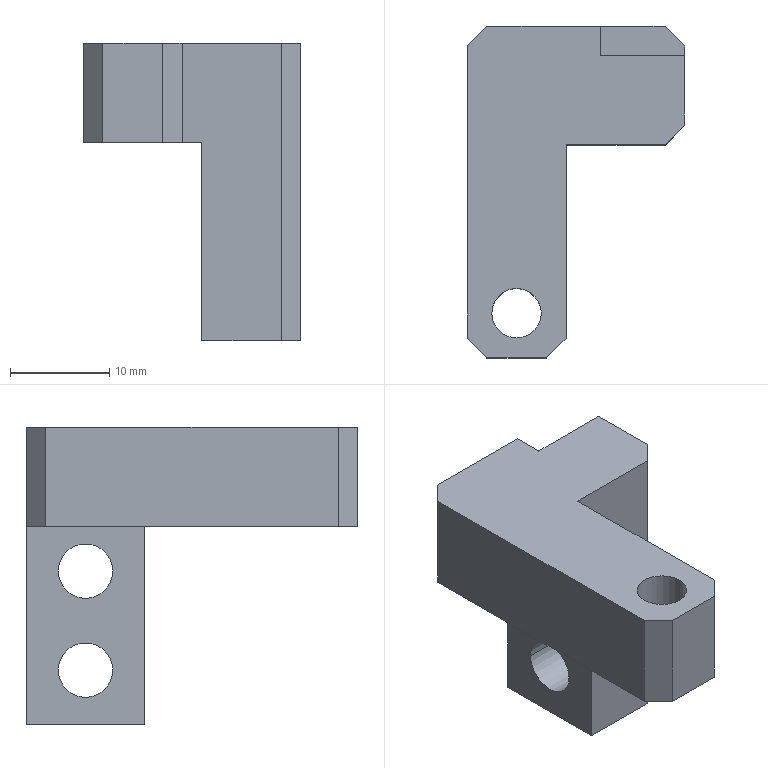Component | SolidWorks | LSDH-6-028-1 | 1 solid | 24 faces | box 22 x 33.5 x 30 mm | volume 6149 mm3 | plane 18 | cylinder 6 | commonest cylinder face diameters 5.5 x4 5 x2
STEP:
#1=COLOUR_RGB('',0.7922,0.8196,0.9333);
#2=FILL_AREA_STYLE_COLOUR('',#1);
#3=FILL_AREA_STYLE('',(#2));
#4=SURFACE_STYLE_FILL_AREA(#3);
#5=SURFACE_SIDE_STYLE('',(#4));
#6=SURFACE_STYLE_USAGE(.BOTH.,#5);
#7=PRESENTATION_STYLE_ASSIGNMENT((#6));
#8=CARTESIAN_POINT('',(10.622,11.897,2.932));
#9=VERTEX_POINT('',#8);
#10=CARTESIAN_POINT('',(10.819,11.897,2.932));
#11=VERTEX_POINT('',#10);
#12=CARTESIAN_POINT('',(10.721,11.897,2.932));
#13=DIRECTION('',(-0.,0.,1.));
#14=DIRECTION('',(0.,1.,0.));
#15=AXIS2_PLACEMENT_3D('',#12,#13,#14);
#16=CIRCLE('',#15,0.09843);
#17=EDGE_CURVE('',#9,#11,#16,.T.);
#18=ORIENTED_EDGE('',*,*,#17,.F.);
#19=CARTESIAN_POINT('',(10.622,11.897,3.326));
#20=VERTEX_POINT('',#19);
#21=CARTESIAN_POINT('',(10.622,11.897,3.326));
#22=DIRECTION('',(-0.,0.,1.));
#23=VECTOR('',#22,39.37);
#24=LINE('',#21,#23);
#25=EDGE_CURVE('',#9,#20,#24,.T.);
#26=ORIENTED_EDGE('',*,*,#25,.T.);
#27=CARTESIAN_POINT('',(10.819,11.897,3.326));
#28=VERTEX_POINT('',#27);
#29=CARTESIAN_POINT('',(10.721,11.897,3.326));
#30=DIRECTION('',(-0.,0.,1.));
#31=DIRECTION('',(1.,0.,0.));
#32=AXIS2_PLACEMENT_3D('',#29,#30,#31);
#33=CIRCLE('',#32,0.09843);
#34=EDGE_CURVE('',#20,#28,#33,.T.);
#35=ORIENTED_EDGE('',*,*,#34,.T.);
#36=CARTESIAN_POINT('',(10.819,11.897,3.326));
#37=DIRECTION('',(-0.,0.,1.));
#38=VECTOR('',#37,39.37);
#39=LINE('',#36,#38);
#40=EDGE_CURVE('',#11,#28,#39,.T.);
#41=ORIENTED_EDGE('',*,*,#40,.F.);
#42=EDGE_LOOP('',(#18,#26,#35,#41));
#43=FACE_OUTER_BOUND('',#42,.T.);
#44=CARTESIAN_POINT('',(10.721,11.897,3.326));
#45=DIRECTION('',(-0.,0.,1.));
#46=DIRECTION('',(1.,0.,0.));
#47=AXIS2_PLACEMENT_3D('',#44,#45,#46);
#48=CYLINDRICAL_SURFACE('',#47,0.09843);
#49=ADVANCED_FACE('',(#43),#48,.F.);
#50=CARTESIAN_POINT('',(11.39,12.694,2.755));
#51=VERTEX_POINT('',#50);
#52=CARTESIAN_POINT('',(11.39,12.91,2.755));
#53=VERTEX_POINT('',#52);
#54=CARTESIAN_POINT('',(11.39,12.802,2.755));
#55=DIRECTION('',(-1.,0.,-0.));
#56=DIRECTION('',(0.,1.,0.));
#57=AXIS2_PLACEMENT_3D('',#54,#55,#56);
#58=CIRCLE('',#57,0.1083);
#59=EDGE_CURVE('',#51,#53,#58,.T.);
#60=ORIENTED_EDGE('',*,*,#59,.F.);
#61=CARTESIAN_POINT('',(10.996,12.694,2.755));
#62=VERTEX_POINT('',#61);
#63=CARTESIAN_POINT('',(10.996,12.694,2.755));
#64=DIRECTION('',(-1.,0.,-0.));
#65=VECTOR('',#64,39.37);
#66=LINE('',#63,#65);
#67=EDGE_CURVE('',#51,#62,#66,.T.);
#68=ORIENTED_EDGE('',*,*,#67,.T.);
#69=CARTESIAN_POINT('',(10.996,12.91,2.755));
#70=VERTEX_POINT('',#69);
#71=CARTESIAN_POINT('',(10.996,12.802,2.755));
#72=DIRECTION('',(-1.,0.,-0.));
#73=DIRECTION('',(0.,1.,0.));
#74=AXIS2_PLACEMENT_3D('',#71,#72,#73);
#75=CIRCLE('',#74,0.1083);
#76=EDGE_CURVE('',#62,#70,#75,.T.);
#77=ORIENTED_EDGE('',*,*,#76,.T.);
#78=CARTESIAN_POINT('',(10.996,12.91,2.755));
#79=DIRECTION('',(-1.,0.,-0.));
#80=VECTOR('',#79,39.37);
#81=LINE('',#78,#80);
#82=EDGE_CURVE('',#53,#70,#81,.T.);
#83=ORIENTED_EDGE('',*,*,#82,.F.);
#84=EDGE_LOOP('',(#60,#68,#77,#83));
#85=FACE_OUTER_BOUND('',#84,.T.);
#86=CARTESIAN_POINT('',(10.996,12.802,2.755));
#87=DIRECTION('',(-1.,0.,-0.));
#88=DIRECTION('',(0.,1.,0.));
#89=AXIS2_PLACEMENT_3D('',#86,#87,#88);
#90=CYLINDRICAL_SURFACE('',#89,0.1083);
#91=ADVANCED_FACE('',(#85),#90,.F.);
#92=CARTESIAN_POINT('',(11.39,12.694,2.361));
#93=VERTEX_POINT('',#92);
#94=CARTESIAN_POINT('',(11.39,12.91,2.361));
#95=VERTEX_POINT('',#94);
#96=CARTESIAN_POINT('',(11.39,12.802,2.361));
#97=DIRECTION('',(-1.,0.,-0.));
#98=DIRECTION('',(0.,1.,0.));
#99=AXIS2_PLACEMENT_3D('',#96,#97,#98);
#100=CIRCLE('',#99,0.1083);
#101=EDGE_CURVE('',#93,#95,#100,.T.);
#102=ORIENTED_EDGE('',*,*,#101,.F.);
#103=CARTESIAN_POINT('',(10.996,12.694,2.361));
#104=VERTEX_POINT('',#103);
#105=CARTESIAN_POINT('',(10.996,12.694,2.361));
#106=DIRECTION('',(-1.,0.,-0.));
#107=VECTOR('',#106,39.37);
#108=LINE('',#105,#107);
#109=EDGE_CURVE('',#93,#104,#108,.T.);
#110=ORIENTED_EDGE('',*,*,#109,.T.);
#111=CARTESIAN_POINT('',(10.996,12.91,2.361));
#112=VERTEX_POINT('',#111);
#113=CARTESIAN_POINT('',(10.996,12.802,2.361));
#114=DIRECTION('',(-1.,0.,-0.));
#115=DIRECTION('',(0.,1.,0.));
#116=AXIS2_PLACEMENT_3D('',#113,#114,#115);
#117=CIRCLE('',#116,0.1083);
#118=EDGE_CURVE('',#104,#112,#117,.T.);
#119=ORIENTED_EDGE('',*,*,#118,.T.);
#120=CARTESIAN_POINT('',(10.996,12.91,2.361));
#121=DIRECTION('',(-1.,0.,-0.));
#122=VECTOR('',#121,39.37);
#123=LINE('',#120,#122);
#124=EDGE_CURVE('',#95,#112,#123,.T.);
#125=ORIENTED_EDGE('',*,*,#124,.F.);
#126=EDGE_LOOP('',(#102,#110,#119,#125));
#127=FACE_OUTER_BOUND('',#126,.T.);
#128=CARTESIAN_POINT('',(10.996,12.802,2.361));
#129=DIRECTION('',(-1.,0.,-0.));
#130=DIRECTION('',(0.,1.,0.));
#131=AXIS2_PLACEMENT_3D('',#128,#129,#130);
#132=CYLINDRICAL_SURFACE('',#131,0.1083);
#133=ADVANCED_FACE('',(#127),#132,.F.);
#134=CARTESIAN_POINT('',(10.996,12.566,2.145));
#135=VERTEX_POINT('',#134);
#136=CARTESIAN_POINT('',(11.311,12.566,2.145));
#137=VERTEX_POINT('',#136);
#138=CARTESIAN_POINT('',(10.996,12.566,2.145));
#139=DIRECTION('',(1.,0.,0.));
#140=VECTOR('',#139,39.37);
#141=LINE('',#138,#140);
#142=EDGE_CURVE('',#135,#137,#141,.T.);
#143=ORIENTED_EDGE('',*,*,#142,.T.);
#144=CARTESIAN_POINT('',(11.311,12.566,3.326));
#145=VERTEX_POINT('',#144);
#146=CARTESIAN_POINT('',(11.311,12.566,2.145));
#147=DIRECTION('',(-0.,0.,1.));
#148=VECTOR('',#147,39.37);
#149=LINE('',#146,#148);
#150=EDGE_CURVE('',#137,#145,#149,.T.);
#151=ORIENTED_EDGE('',*,*,#150,.T.);
#152=CARTESIAN_POINT('',(10.918,12.566,3.326));
#153=VERTEX_POINT('',#152);
#154=CARTESIAN_POINT('',(10.996,12.566,3.326));
#155=DIRECTION('',(1.,0.,0.));
#156=VECTOR('',#155,39.37);
#157=LINE('',#154,#156);
#158=EDGE_CURVE('',#153,#145,#157,.T.);
#159=ORIENTED_EDGE('',*,*,#158,.F.);
#160=CARTESIAN_POINT('',(10.918,12.566,2.932));
#161=VERTEX_POINT('',#160);
#162=CARTESIAN_POINT('',(10.918,12.566,3.326));
#163=DIRECTION('',(-0.,0.,1.));
#164=VECTOR('',#163,39.37);
#165=LINE('',#162,#164);
#166=EDGE_CURVE('',#161,#153,#165,.T.);
#167=ORIENTED_EDGE('',*,*,#166,.F.);
#168=CARTESIAN_POINT('',(10.996,12.566,2.932));
#169=VERTEX_POINT('',#168);
#170=CARTESIAN_POINT('',(10.524,12.566,2.932));
#171=DIRECTION('',(1.,0.,0.));
#172=VECTOR('',#171,39.37);
#173=LINE('',#170,#172);
#174=EDGE_CURVE('',#161,#169,#173,.T.);
#175=ORIENTED_EDGE('',*,*,#174,.T.);
#176=CARTESIAN_POINT('',(10.996,12.566,2.145));
#177=DIRECTION('',(-0.,0.,1.));
#178=VECTOR('',#177,39.37);
#179=LINE('',#176,#178);
#180=EDGE_CURVE('',#135,#169,#179,.T.);
#181=ORIENTED_EDGE('',*,*,#180,.F.);
#182=EDGE_LOOP('',(#143,#151,#159,#167,#175,#181));
#183=FACE_OUTER_BOUND('',#182,.T.);
#184=CARTESIAN_POINT('',(10.996,12.566,2.145));
#185=DIRECTION('',(0.,1.,-0.));
#186=DIRECTION('',(0.,-0.,-1.));
#187=AXIS2_PLACEMENT_3D('',#184,#185,#186);
#188=PLANE('',#187);
#189=ADVANCED_FACE('',(#183),#188,.F.);
#190=CARTESIAN_POINT('',(11.054,13.038,3.326));
#191=VERTEX_POINT('',#190);
#192=CARTESIAN_POINT('',(10.603,13.038,3.326));
#193=VERTEX_POINT('',#192);
#194=CARTESIAN_POINT('',(10.996,13.038,3.326));
#195=DIRECTION('',(-1.,-0.,-0.));
#196=VECTOR('',#195,39.37);
#197=LINE('',#194,#196);
#198=EDGE_CURVE('',#191,#193,#197,.T.);
#199=ORIENTED_EDGE('',*,*,#198,.F.);
#200=CARTESIAN_POINT('',(11.054,13.038,3.011));
#201=VERTEX_POINT('',#200);
#202=CARTESIAN_POINT('',(11.054,13.038,3.326));
#203=DIRECTION('',(-0.,0.,1.));
#204=VECTOR('',#203,39.37);
#205=LINE('',#202,#204);
#206=EDGE_CURVE('',#201,#191,#205,.T.);
#207=ORIENTED_EDGE('',*,*,#206,.F.);
#208=CARTESIAN_POINT('',(11.311,13.038,3.011));
#209=VERTEX_POINT('',#208);
#210=CARTESIAN_POINT('',(11.054,13.038,3.011));
#211=DIRECTION('',(-1.,0.,-0.));
#212=VECTOR('',#211,39.37);
#213=LINE('',#210,#212);
#214=EDGE_CURVE('',#209,#201,#213,.T.);
#215=ORIENTED_EDGE('',*,*,#214,.F.);
#216=CARTESIAN_POINT('',(11.311,13.038,2.145));
#217=VERTEX_POINT('',#216);
#218=CARTESIAN_POINT('',(11.311,13.038,2.145));
#219=DIRECTION('',(0.,-0.,-1.));
#220=VECTOR('',#219,39.37);
#221=LINE('',#218,#220);
#222=EDGE_CURVE('',#209,#217,#221,.T.);
#223=ORIENTED_EDGE('',*,*,#222,.T.);
#224=CARTESIAN_POINT('',(10.996,13.038,2.145));
#225=VERTEX_POINT('',#224);
#226=CARTESIAN_POINT('',(10.996,13.038,2.145));
#227=DIRECTION('',(1.,0.,0.));
#228=VECTOR('',#227,39.37);
#229=LINE('',#226,#228);
#230=EDGE_CURVE('',#225,#217,#229,.T.);
#231=ORIENTED_EDGE('',*,*,#230,.F.);
#232=CARTESIAN_POINT('',(10.996,13.038,2.932));
#233=VERTEX_POINT('',#232);
#234=CARTESIAN_POINT('',(10.996,13.038,2.145));
#235=DIRECTION('',(0.,-0.,-1.));
#236=VECTOR('',#235,39.37);
#237=LINE('',#234,#236);
#238=EDGE_CURVE('',#233,#225,#237,.T.);
#239=ORIENTED_EDGE('',*,*,#238,.F.);
#240=CARTESIAN_POINT('',(10.603,13.038,2.932));
#241=VERTEX_POINT('',#240);
#242=CARTESIAN_POINT('',(10.524,13.038,2.932));
#243=DIRECTION('',(1.,0.,0.));
#244=VECTOR('',#243,39.37);
#245=LINE('',#242,#244);
#246=EDGE_CURVE('',#241,#233,#245,.T.);
#247=ORIENTED_EDGE('',*,*,#246,.F.);
#248=CARTESIAN_POINT('',(10.603,13.038,3.326));
#249=DIRECTION('',(-0.,0.,1.));
#250=VECTOR('',#249,39.37);
#251=LINE('',#248,#250);
#252=EDGE_CURVE('',#241,#193,#251,.T.);
#253=ORIENTED_EDGE('',*,*,#252,.T.);
#254=EDGE_LOOP('',(#199,#207,#215,#223,#231,#239,#247,#253));
#255=FACE_OUTER_BOUND('',#254,.T.);
#256=CARTESIAN_POINT('',(10.996,13.038,2.145));
#257=DIRECTION('',(-0.,-1.,0.));
#258=DIRECTION('',(-0.,0.,1.));
#259=AXIS2_PLACEMENT_3D('',#256,#257,#258);
#260=PLANE('',#259);
#261=ADVANCED_FACE('',(#255),#260,.F.);
#262=ORIENTED_EDGE('',*,*,#230,.T.);
#263=CARTESIAN_POINT('',(11.39,12.96,2.145));
#264=VERTEX_POINT('',#263);
#265=CARTESIAN_POINT('',(11.311,13.038,2.145));
#266=DIRECTION('',(0.7071,-0.7071,0.));
#267=VECTOR('',#266,39.37);
#268=LINE('',#265,#267);
#269=EDGE_CURVE('',#217,#264,#268,.T.);
#270=ORIENTED_EDGE('',*,*,#269,.T.);
#271=CARTESIAN_POINT('',(11.39,12.645,2.145));
#272=VERTEX_POINT('',#271);
#273=CARTESIAN_POINT('',(11.39,12.566,2.145));
#274=DIRECTION('',(0.,-1.,0.));
#275=VECTOR('',#274,39.37);
#276=LINE('',#273,#275);
#277=EDGE_CURVE('',#264,#272,#276,.T.);
#278=ORIENTED_EDGE('',*,*,#277,.T.);
#279=CARTESIAN_POINT('',(11.311,12.566,2.145));
#280=DIRECTION('',(-0.7071,-0.7071,-0.));
#281=VECTOR('',#280,39.37);
#282=LINE('',#279,#281);
#283=EDGE_CURVE('',#272,#137,#282,.T.);
#284=ORIENTED_EDGE('',*,*,#283,.T.);
#285=ORIENTED_EDGE('',*,*,#142,.F.);
#286=CARTESIAN_POINT('',(10.996,12.566,2.145));
#287=DIRECTION('',(0.,-1.,0.));
#288=VECTOR('',#287,39.37);
#289=LINE('',#286,#288);
#290=EDGE_CURVE('',#225,#135,#289,.T.);
#291=ORIENTED_EDGE('',*,*,#290,.F.);
#292=EDGE_LOOP('',(#262,#270,#278,#284,#285,#291));
#293=FACE_OUTER_BOUND('',#292,.T.);
#294=CARTESIAN_POINT('',(10.996,12.566,2.145));
#295=DIRECTION('',(-0.,0.,1.));
#296=DIRECTION('',(1.,0.,0.));
#297=AXIS2_PLACEMENT_3D('',#294,#295,#296);
#298=PLANE('',#297);
#299=ADVANCED_FACE('',(#293),#298,.F.);
#300=CARTESIAN_POINT('',(10.996,13.038,2.932));
#301=DIRECTION('',(-0.,-1.,0.));
#302=VECTOR('',#301,39.37);
#303=LINE('',#300,#302);
#304=EDGE_CURVE('',#233,#169,#303,.T.);
#305=ORIENTED_EDGE('',*,*,#304,.F.);
#306=ORIENTED_EDGE('',*,*,#238,.T.);
#307=ORIENTED_EDGE('',*,*,#290,.T.);
#308=ORIENTED_EDGE('',*,*,#180,.T.);
#309=EDGE_LOOP('',(#305,#306,#307,#308));
#310=FACE_OUTER_BOUND('',#309,.T.);
#311=CARTESIAN_POINT('',(10.996,12.802,2.755));
#312=DIRECTION('',(-1.,0.,-0.));
#313=DIRECTION('',(0.,1.,0.));
#314=AXIS2_PLACEMENT_3D('',#311,#312,#313);
#315=CIRCLE('',#314,0.1083);
#316=EDGE_CURVE('',#70,#62,#315,.T.);
#317=ORIENTED_EDGE('',*,*,#316,.F.);
#318=ORIENTED_EDGE('',*,*,#76,.F.);
#319=EDGE_LOOP('',(#317,#318));
#320=FACE_BOUND('',#319,.T.);
#321=CARTESIAN_POINT('',(10.996,12.802,2.361));
#322=DIRECTION('',(-1.,0.,-0.));
#323=DIRECTION('',(0.,1.,0.));
#324=AXIS2_PLACEMENT_3D('',#321,#322,#323);
#325=CIRCLE('',#324,0.1083);
#326=EDGE_CURVE('',#112,#104,#325,.T.);
#327=ORIENTED_EDGE('',*,*,#326,.F.);
#328=ORIENTED_EDGE('',*,*,#118,.F.);
#329=EDGE_LOOP('',(#327,#328));
#330=FACE_BOUND('',#329,.T.);
#331=CARTESIAN_POINT('',(10.996,12.566,2.145));
#332=DIRECTION('',(-1.,0.,-0.));
#333=DIRECTION('',(0.,1.,0.));
#334=AXIS2_PLACEMENT_3D('',#331,#332,#333);
#335=PLANE('',#334);
#336=ADVANCED_FACE('',(#310,#320,#330),#335,.T.);
#337=CARTESIAN_POINT('',(11.39,12.802,2.755));
#338=DIRECTION('',(-1.,0.,-0.));
#339=DIRECTION('',(0.,1.,0.));
#340=AXIS2_PLACEMENT_3D('',#337,#338,#339);
#341=CIRCLE('',#340,0.1083);
#342=EDGE_CURVE('',#53,#51,#341,.T.);
#343=ORIENTED_EDGE('',*,*,#342,.T.);
#344=ORIENTED_EDGE('',*,*,#59,.T.);
#345=EDGE_LOOP('',(#343,#344));
#346=FACE_BOUND('',#345,.T.);
#347=CARTESIAN_POINT('',(11.39,12.802,2.361));
#348=DIRECTION('',(-1.,0.,-0.));
#349=DIRECTION('',(0.,1.,0.));
#350=AXIS2_PLACEMENT_3D('',#347,#348,#349);
#351=CIRCLE('',#350,0.1083);
#352=EDGE_CURVE('',#95,#93,#351,.T.);
#353=ORIENTED_EDGE('',*,*,#352,.T.);
#354=ORIENTED_EDGE('',*,*,#101,.T.);
#355=EDGE_LOOP('',(#353,#354));
#356=FACE_BOUND('',#355,.T.);
#357=CARTESIAN_POINT('',(11.39,12.96,3.011));
#358=VERTEX_POINT('',#357);
#359=CARTESIAN_POINT('',(11.39,12.96,2.145));
#360=DIRECTION('',(-0.,0.,1.));
#361=VECTOR('',#360,39.37);
#362=LINE('',#359,#361);
#363=EDGE_CURVE('',#264,#358,#362,.T.);
#364=ORIENTED_EDGE('',*,*,#363,.T.);
#365=CARTESIAN_POINT('',(11.39,12.92,3.011));
#366=VERTEX_POINT('',#365);
#367=CARTESIAN_POINT('',(11.39,12.92,3.011));
#368=DIRECTION('',(0.,1.,-0.));
#369=VECTOR('',#368,39.37);
#370=LINE('',#367,#369);
#371=EDGE_CURVE('',#366,#358,#370,.T.);
#372=ORIENTED_EDGE('',*,*,#371,.F.);
#373=CARTESIAN_POINT('',(11.39,12.92,3.326));
#374=VERTEX_POINT('',#373);
#375=CARTESIAN_POINT('',(11.39,12.92,3.326));
#376=DIRECTION('',(0.,-0.,-1.));
#377=VECTOR('',#376,39.37);
#378=LINE('',#375,#377);
#379=EDGE_CURVE('',#374,#366,#378,.T.);
#380=ORIENTED_EDGE('',*,*,#379,.F.);
#381=CARTESIAN_POINT('',(11.39,12.645,3.326));
#382=VERTEX_POINT('',#381);
#383=CARTESIAN_POINT('',(11.39,12.566,3.326));
#384=DIRECTION('',(0.,1.,0.));
#385=VECTOR('',#384,39.37);
#386=LINE('',#383,#385);
#387=EDGE_CURVE('',#382,#374,#386,.T.);
#388=ORIENTED_EDGE('',*,*,#387,.F.);
#389=CARTESIAN_POINT('',(11.39,12.645,2.145));
#390=DIRECTION('',(0.,-0.,-1.));
#391=VECTOR('',#390,39.37);
#392=LINE('',#389,#391);
#393=EDGE_CURVE('',#382,#272,#392,.T.);
#394=ORIENTED_EDGE('',*,*,#393,.T.);
#395=ORIENTED_EDGE('',*,*,#277,.F.);
#396=EDGE_LOOP('',(#364,#372,#380,#388,#394,#395));
#397=FACE_OUTER_BOUND('',#396,.T.);
#398=CARTESIAN_POINT('',(11.39,12.566,2.145));
#399=DIRECTION('',(-1.,0.,-0.));
#400=DIRECTION('',(0.,1.,0.));
#401=AXIS2_PLACEMENT_3D('',#398,#399,#400);
#402=PLANE('',#401);
#403=ADVANCED_FACE('',(#346,#356,#397),#402,.F.);
#404=ORIENTED_EDGE('',*,*,#109,.F.);
#405=ORIENTED_EDGE('',*,*,#352,.F.);
#406=ORIENTED_EDGE('',*,*,#124,.T.);
#407=ORIENTED_EDGE('',*,*,#326,.T.);
#408=EDGE_LOOP('',(#404,#405,#406,#407));
#409=FACE_OUTER_BOUND('',#408,.T.);
#410=CARTESIAN_POINT('',(10.996,12.802,2.361));
#411=DIRECTION('',(-1.,0.,-0.));
#412=DIRECTION('',(0.,1.,0.));
#413=AXIS2_PLACEMENT_3D('',#410,#411,#412);
#414=CYLINDRICAL_SURFACE('',#413,0.1083);
#415=ADVANCED_FACE('',(#409),#414,.F.);
#416=ORIENTED_EDGE('',*,*,#67,.F.);
#417=ORIENTED_EDGE('',*,*,#342,.F.);
#418=ORIENTED_EDGE('',*,*,#82,.T.);
#419=ORIENTED_EDGE('',*,*,#316,.T.);
#420=EDGE_LOOP('',(#416,#417,#418,#419));
#421=FACE_OUTER_BOUND('',#420,.T.);
#422=CARTESIAN_POINT('',(10.996,12.802,2.755));
#423=DIRECTION('',(-1.,0.,-0.));
#424=DIRECTION('',(0.,1.,0.));
#425=AXIS2_PLACEMENT_3D('',#422,#423,#424);
#426=CYLINDRICAL_SURFACE('',#425,0.1083);
#427=ADVANCED_FACE('',(#421),#426,.F.);
#428=CARTESIAN_POINT('',(11.054,12.92,3.326));
#429=VERTEX_POINT('',#428);
#430=CARTESIAN_POINT('',(11.054,12.92,3.326));
#431=DIRECTION('',(0.,1.,-0.));
#432=VECTOR('',#431,39.37);
#433=LINE('',#430,#432);
#434=EDGE_CURVE('',#429,#191,#433,.T.);
#435=ORIENTED_EDGE('',*,*,#434,.T.);
#436=ORIENTED_EDGE('',*,*,#198,.T.);
#437=CARTESIAN_POINT('',(10.524,12.96,3.326));
#438=VERTEX_POINT('',#437);
#439=CARTESIAN_POINT('',(10.76,13.196,3.326));
#440=DIRECTION('',(-0.7071,-0.7071,-0.));
#441=VECTOR('',#440,39.37);
#442=LINE('',#439,#441);
#443=EDGE_CURVE('',#193,#438,#442,.T.);
#444=ORIENTED_EDGE('',*,*,#443,.T.);
#445=CARTESIAN_POINT('',(10.524,11.798,3.326));
#446=VERTEX_POINT('',#445);
#447=CARTESIAN_POINT('',(10.524,13.038,3.326));
#448=DIRECTION('',(0.,1.,0.));
#449=VECTOR('',#448,39.37);
#450=LINE('',#447,#449);
#451=EDGE_CURVE('',#446,#438,#450,.T.);
#452=ORIENTED_EDGE('',*,*,#451,.F.);
#453=CARTESIAN_POINT('',(10.603,11.72,3.326));
#454=VERTEX_POINT('',#453);
#455=CARTESIAN_POINT('',(10.573,11.749,3.326));
#456=DIRECTION('',(0.7071,-0.7071,0.));
#457=VECTOR('',#456,39.37);
#458=LINE('',#455,#457);
#459=EDGE_CURVE('',#446,#454,#458,.T.);
#460=ORIENTED_EDGE('',*,*,#459,.T.);
#461=CARTESIAN_POINT('',(10.839,11.72,3.326));
#462=VERTEX_POINT('',#461);
#463=CARTESIAN_POINT('',(10.524,11.72,3.326));
#464=DIRECTION('',(-1.,0.,-0.));
#465=VECTOR('',#464,39.37);
#466=LINE('',#463,#465);
#467=EDGE_CURVE('',#462,#454,#466,.T.);
#468=ORIENTED_EDGE('',*,*,#467,.F.);
#469=CARTESIAN_POINT('',(10.918,11.798,3.326));
#470=VERTEX_POINT('',#469);
#471=CARTESIAN_POINT('',(11.538,12.418,3.326));
#472=DIRECTION('',(0.7071,0.7071,0.));
#473=VECTOR('',#472,39.37);
#474=LINE('',#471,#473);
#475=EDGE_CURVE('',#462,#470,#474,.T.);
#476=ORIENTED_EDGE('',*,*,#475,.T.);
#477=CARTESIAN_POINT('',(10.918,11.72,3.326));
#478=DIRECTION('',(0.,1.,-0.));
#479=VECTOR('',#478,39.37);
#480=LINE('',#477,#479);
#481=EDGE_CURVE('',#470,#153,#480,.T.);
#482=ORIENTED_EDGE('',*,*,#481,.T.);
#483=ORIENTED_EDGE('',*,*,#158,.T.);
#484=CARTESIAN_POINT('',(11.351,12.605,3.326));
#485=DIRECTION('',(0.7071,0.7071,0.));
#486=VECTOR('',#485,39.37);
#487=LINE('',#484,#486);
#488=EDGE_CURVE('',#145,#382,#487,.T.);
#489=ORIENTED_EDGE('',*,*,#488,.T.);
#490=ORIENTED_EDGE('',*,*,#387,.T.);
#491=CARTESIAN_POINT('',(11.054,12.92,3.326));
#492=DIRECTION('',(1.,0.,0.));
#493=VECTOR('',#492,39.37);
#494=LINE('',#491,#493);
#495=EDGE_CURVE('',#429,#374,#494,.T.);
#496=ORIENTED_EDGE('',*,*,#495,.F.);
#497=EDGE_LOOP('',(#435,#436,#444,#452,#460,#468,#476,#482,#483,#489,#490,#496));
#498=FACE_OUTER_BOUND('',#497,.T.);
#499=CARTESIAN_POINT('',(10.721,11.897,3.326));
#500=DIRECTION('',(-0.,0.,1.));
#501=DIRECTION('',(1.,0.,0.));
#502=AXIS2_PLACEMENT_3D('',#499,#500,#501);
#503=CIRCLE('',#502,0.09843);
#504=EDGE_CURVE('',#28,#20,#503,.T.);
#505=ORIENTED_EDGE('',*,*,#504,.F.);
#506=ORIENTED_EDGE('',*,*,#34,.F.);
#507=EDGE_LOOP('',(#505,#506));
#508=FACE_BOUND('',#507,.T.);
#509=CARTESIAN_POINT('',(11.39,12.566,3.326));
#510=DIRECTION('',(-0.,0.,1.));
#511=DIRECTION('',(1.,0.,0.));
#512=AXIS2_PLACEMENT_3D('',#509,#510,#511);
#513=PLANE('',#512);
#514=ADVANCED_FACE('',(#498,#508),#513,.T.);
#515=CARTESIAN_POINT('',(10.721,11.897,2.932));
#516=DIRECTION('',(-0.,0.,1.));
#517=DIRECTION('',(0.,1.,0.));
#518=AXIS2_PLACEMENT_3D('',#515,#516,#517);
#519=CIRCLE('',#518,0.09843);
#520=EDGE_CURVE('',#11,#9,#519,.T.);
#521=ORIENTED_EDGE('',*,*,#520,.T.);
#522=ORIENTED_EDGE('',*,*,#17,.T.);
#523=EDGE_LOOP('',(#521,#522));
#524=FACE_BOUND('',#523,.T.);
#525=CARTESIAN_POINT('',(10.524,12.96,2.932));
#526=VERTEX_POINT('',#525);
#527=CARTESIAN_POINT('',(10.524,11.798,2.932));
#528=VERTEX_POINT('',#527);
#529=CARTESIAN_POINT('',(10.524,13.038,2.932));
#530=DIRECTION('',(-0.,-1.,0.));
#531=VECTOR('',#530,39.37);
#532=LINE('',#529,#531);
#533=EDGE_CURVE('',#526,#528,#532,.T.);
#534=ORIENTED_EDGE('',*,*,#533,.F.);
#535=CARTESIAN_POINT('',(10.524,12.96,2.932));
#536=DIRECTION('',(0.7071,0.7071,-0.));
#537=VECTOR('',#536,39.37);
#538=LINE('',#535,#537);
#539=EDGE_CURVE('',#526,#241,#538,.T.);
#540=ORIENTED_EDGE('',*,*,#539,.T.);
#541=ORIENTED_EDGE('',*,*,#246,.T.);
#542=ORIENTED_EDGE('',*,*,#304,.T.);
#543=ORIENTED_EDGE('',*,*,#174,.F.);
#544=CARTESIAN_POINT('',(10.918,11.798,2.932));
#545=VERTEX_POINT('',#544);
#546=CARTESIAN_POINT('',(10.918,11.72,2.932));
#547=DIRECTION('',(0.,1.,-0.));
#548=VECTOR('',#547,39.37);
#549=LINE('',#546,#548);
#550=EDGE_CURVE('',#545,#161,#549,.T.);
#551=ORIENTED_EDGE('',*,*,#550,.F.);
#552=CARTESIAN_POINT('',(10.839,11.72,2.932));
#553=VERTEX_POINT('',#552);
#554=CARTESIAN_POINT('',(10.839,11.72,2.932));
#555=DIRECTION('',(-0.7071,-0.7071,0.));
#556=VECTOR('',#555,39.37);
#557=LINE('',#554,#556);
#558=EDGE_CURVE('',#545,#553,#557,.T.);
#559=ORIENTED_EDGE('',*,*,#558,.T.);
#560=CARTESIAN_POINT('',(10.603,11.72,2.932));
#561=VERTEX_POINT('',#560);
#562=CARTESIAN_POINT('',(10.524,11.72,2.932));
#563=DIRECTION('',(1.,0.,0.));
#564=VECTOR('',#563,39.37);
#565=LINE('',#562,#564);
#566=EDGE_CURVE('',#561,#553,#565,.T.);
#567=ORIENTED_EDGE('',*,*,#566,.F.);
#568=CARTESIAN_POINT('',(10.603,11.72,2.932));
#569=DIRECTION('',(-0.7071,0.7071,-0.));
#570=VECTOR('',#569,39.37);
#571=LINE('',#568,#570);
#572=EDGE_CURVE('',#561,#528,#571,.T.);
#573=ORIENTED_EDGE('',*,*,#572,.T.);
#574=EDGE_LOOP('',(#534,#540,#541,#542,#543,#551,#559,#567,#573));
#575=FACE_OUTER_BOUND('',#574,.T.);
#576=CARTESIAN_POINT('',(10.524,13.038,2.932));
#577=DIRECTION('',(-0.,0.,1.));
#578=DIRECTION('',(0.,1.,-0.));
#579=AXIS2_PLACEMENT_3D('',#576,#577,#578);
#580=PLANE('',#579);
#581=ADVANCED_FACE('',(#524,#575),#580,.F.);
#582=ORIENTED_EDGE('',*,*,#451,.T.);
#583=CARTESIAN_POINT('',(10.524,12.96,2.932));
#584=DIRECTION('',(0.,-0.,-1.));
#585=VECTOR('',#584,39.37);
#586=LINE('',#583,#585);
#587=EDGE_CURVE('',#438,#526,#586,.T.);
#588=ORIENTED_EDGE('',*,*,#587,.T.);
#589=ORIENTED_EDGE('',*,*,#533,.T.);
#590=CARTESIAN_POINT('',(10.524,11.798,2.145));
#591=DIRECTION('',(-0.,0.,1.));
#592=VECTOR('',#591,39.37);
#593=LINE('',#590,#592);
#594=EDGE_CURVE('',#528,#446,#593,.T.);
#595=ORIENTED_EDGE('',*,*,#594,.T.);
#596=EDGE_LOOP('',(#582,#588,#589,#595));
#597=FACE_OUTER_BOUND('',#596,.T.);
#598=CARTESIAN_POINT('',(10.524,12.566,2.145));
#599=DIRECTION('',(-1.,0.,-0.));
#600=DIRECTION('',(0.,1.,0.));
#601=AXIS2_PLACEMENT_3D('',#598,#599,#600);
#602=PLANE('',#601);
#603=ADVANCED_FACE('',(#597),#602,.T.);
#604=ORIENTED_EDGE('',*,*,#481,.F.);
#605=CARTESIAN_POINT('',(10.918,11.798,2.932));
#606=DIRECTION('',(0.,-0.,-1.));
#607=VECTOR('',#606,39.37);
#608=LINE('',#605,#607);
#609=EDGE_CURVE('',#470,#545,#608,.T.);
#610=ORIENTED_EDGE('',*,*,#609,.T.);
#611=ORIENTED_EDGE('',*,*,#550,.T.);
#612=ORIENTED_EDGE('',*,*,#166,.T.);
#613=EDGE_LOOP('',(#604,#610,#611,#612));
#614=FACE_OUTER_BOUND('',#613,.T.);
#615=CARTESIAN_POINT('',(10.918,11.72,3.326));
#616=DIRECTION('',(-1.,0.,-0.));
#617=DIRECTION('',(0.,1.,0.));
#618=AXIS2_PLACEMENT_3D('',#615,#616,#617);
#619=PLANE('',#618);
#620=ADVANCED_FACE('',(#614),#619,.F.);
#621=ORIENTED_EDGE('',*,*,#566,.T.);
#622=CARTESIAN_POINT('',(10.839,11.72,3.326));
#623=DIRECTION('',(-0.,0.,1.));
#624=VECTOR('',#623,39.37);
#625=LINE('',#622,#624);
#626=EDGE_CURVE('',#553,#462,#625,.T.);
#627=ORIENTED_EDGE('',*,*,#626,.T.);
#628=ORIENTED_EDGE('',*,*,#467,.T.);
#629=CARTESIAN_POINT('',(10.603,11.72,2.145));
#630=DIRECTION('',(0.,-0.,-1.));
#631=VECTOR('',#630,39.37);
#632=LINE('',#629,#631);
#633=EDGE_CURVE('',#454,#561,#632,.T.);
#634=ORIENTED_EDGE('',*,*,#633,.T.);
#635=EDGE_LOOP('',(#621,#627,#628,#634));
#636=FACE_OUTER_BOUND('',#635,.T.);
#637=CARTESIAN_POINT('',(11.39,11.72,2.145));
#638=DIRECTION('',(-0.,-1.,0.));
#639=DIRECTION('',(-0.,0.,1.));
#640=AXIS2_PLACEMENT_3D('',#637,#638,#639);
#641=PLANE('',#640);
#642=ADVANCED_FACE('',(#636),#641,.T.);
#643=ORIENTED_EDGE('',*,*,#25,.F.);
#644=ORIENTED_EDGE('',*,*,#520,.F.);
#645=ORIENTED_EDGE('',*,*,#40,.T.);
#646=ORIENTED_EDGE('',*,*,#504,.T.);
#647=EDGE_LOOP('',(#643,#644,#645,#646));
#648=FACE_OUTER_BOUND('',#647,.T.);
#649=CARTESIAN_POINT('',(10.721,11.897,3.326));
#650=DIRECTION('',(-0.,0.,1.));
#651=DIRECTION('',(1.,0.,0.));
#652=AXIS2_PLACEMENT_3D('',#649,#650,#651);
#653=CYLINDRICAL_SURFACE('',#652,0.09843);
#654=ADVANCED_FACE('',(#648),#653,.F.);
#655=ORIENTED_EDGE('',*,*,#443,.F.);
#656=ORIENTED_EDGE('',*,*,#252,.F.);
#657=ORIENTED_EDGE('',*,*,#539,.F.);
#658=ORIENTED_EDGE('',*,*,#587,.F.);
#659=EDGE_LOOP('',(#655,#656,#657,#658));
#660=FACE_OUTER_BOUND('',#659,.T.);
#661=CARTESIAN_POINT('',(10.524,12.96,2.145));
#662=DIRECTION('',(-0.7071,0.7071,-0.));
#663=DIRECTION('',(-0.,0.,1.));
#664=AXIS2_PLACEMENT_3D('',#661,#662,#663);
#665=PLANE('',#664);
#666=ADVANCED_FACE('',(#660),#665,.T.);
#667=CARTESIAN_POINT('',(11.311,13.038,3.011));
#668=DIRECTION('',(-0.7071,0.7071,-0.));
#669=VECTOR('',#668,39.37);
#670=LINE('',#667,#669);
#671=EDGE_CURVE('',#358,#209,#670,.T.);
#672=ORIENTED_EDGE('',*,*,#671,.F.);
#673=ORIENTED_EDGE('',*,*,#363,.F.);
#674=ORIENTED_EDGE('',*,*,#269,.F.);
#675=ORIENTED_EDGE('',*,*,#222,.F.);
#676=EDGE_LOOP('',(#672,#673,#674,#675));
#677=FACE_OUTER_BOUND('',#676,.T.);
#678=CARTESIAN_POINT('',(11.311,13.038,2.145));
#679=DIRECTION('',(-0.7071,-0.7071,-0.));
#680=DIRECTION('',(0.,-0.,-1.));
#681=AXIS2_PLACEMENT_3D('',#678,#679,#680);
#682=PLANE('',#681);
#683=ADVANCED_FACE('',(#677),#682,.F.);
#684=ORIENTED_EDGE('',*,*,#283,.F.);
#685=ORIENTED_EDGE('',*,*,#393,.F.);
#686=ORIENTED_EDGE('',*,*,#488,.F.);
#687=ORIENTED_EDGE('',*,*,#150,.F.);
#688=EDGE_LOOP('',(#684,#685,#686,#687));
#689=FACE_OUTER_BOUND('',#688,.T.);
#690=CARTESIAN_POINT('',(11.311,12.566,2.145));
#691=DIRECTION('',(-0.7071,0.7071,-0.));
#692=DIRECTION('',(-0.,0.,1.));
#693=AXIS2_PLACEMENT_3D('',#690,#691,#692);
#694=PLANE('',#693);
#695=ADVANCED_FACE('',(#689),#694,.F.);
#696=ORIENTED_EDGE('',*,*,#558,.F.);
#697=ORIENTED_EDGE('',*,*,#609,.F.);
#698=ORIENTED_EDGE('',*,*,#475,.F.);
#699=ORIENTED_EDGE('',*,*,#626,.F.);
#700=EDGE_LOOP('',(#696,#697,#698,#699));
#701=FACE_OUTER_BOUND('',#700,.T.);
#702=CARTESIAN_POINT('',(10.839,11.72,2.145));
#703=DIRECTION('',(0.7071,-0.7071,0.));
#704=DIRECTION('',(0.,-0.,-1.));
#705=AXIS2_PLACEMENT_3D('',#702,#703,#704);
#706=PLANE('',#705);
#707=ADVANCED_FACE('',(#701),#706,.T.);
#708=ORIENTED_EDGE('',*,*,#459,.F.);
#709=ORIENTED_EDGE('',*,*,#594,.F.);
#710=ORIENTED_EDGE('',*,*,#572,.F.);
#711=ORIENTED_EDGE('',*,*,#633,.F.);
#712=EDGE_LOOP('',(#708,#709,#710,#711));
#713=FACE_OUTER_BOUND('',#712,.T.);
#714=CARTESIAN_POINT('',(10.603,11.72,2.145));
#715=DIRECTION('',(0.7071,0.7071,0.));
#716=DIRECTION('',(0.,-0.,-1.));
#717=AXIS2_PLACEMENT_3D('',#714,#715,#716);
#718=PLANE('',#717);
#719=ADVANCED_FACE('',(#713),#718,.F.);
#720=ORIENTED_EDGE('',*,*,#206,.T.);
#721=ORIENTED_EDGE('',*,*,#434,.F.);
#722=CARTESIAN_POINT('',(11.054,12.92,3.011));
#723=VERTEX_POINT('',#722);
#724=CARTESIAN_POINT('',(11.054,12.92,3.326));
#725=DIRECTION('',(-0.,0.,1.));
#726=VECTOR('',#725,39.37);
#727=LINE('',#724,#726);
#728=EDGE_CURVE('',#723,#429,#727,.T.);
#729=ORIENTED_EDGE('',*,*,#728,.F.);
#730=CARTESIAN_POINT('',(11.054,12.92,3.011));
#731=DIRECTION('',(0.,1.,-0.));
#732=VECTOR('',#731,39.37);
#733=LINE('',#730,#732);
#734=EDGE_CURVE('',#723,#201,#733,.T.);
#735=ORIENTED_EDGE('',*,*,#734,.T.);
#736=EDGE_LOOP('',(#720,#721,#729,#735));
#737=FACE_OUTER_BOUND('',#736,.T.);
#738=CARTESIAN_POINT('',(11.054,12.92,3.326));
#739=DIRECTION('',(-1.,0.,-0.));
#740=DIRECTION('',(0.,1.,0.));
#741=AXIS2_PLACEMENT_3D('',#738,#739,#740);
#742=PLANE('',#741);
#743=ADVANCED_FACE('',(#737),#742,.F.);
#744=ORIENTED_EDGE('',*,*,#671,.T.);
#745=ORIENTED_EDGE('',*,*,#214,.T.);
#746=ORIENTED_EDGE('',*,*,#734,.F.);
#747=CARTESIAN_POINT('',(11.054,12.92,3.011));
#748=DIRECTION('',(-1.,0.,-0.));
#749=VECTOR('',#748,39.37);
#750=LINE('',#747,#749);
#751=EDGE_CURVE('',#366,#723,#750,.T.);
#752=ORIENTED_EDGE('',*,*,#751,.F.);
#753=ORIENTED_EDGE('',*,*,#371,.T.);
#754=EDGE_LOOP('',(#744,#745,#746,#752,#753));
#755=FACE_OUTER_BOUND('',#754,.T.);
#756=CARTESIAN_POINT('',(11.054,12.92,3.011));
#757=DIRECTION('',(0.,-0.,-1.));
#758=DIRECTION('',(-0.,-1.,0.));
#759=AXIS2_PLACEMENT_3D('',#756,#757,#758);
#760=PLANE('',#759);
#761=ADVANCED_FACE('',(#755),#760,.F.);
#762=ORIENTED_EDGE('',*,*,#728,.T.);
#763=ORIENTED_EDGE('',*,*,#495,.T.);
#764=ORIENTED_EDGE('',*,*,#379,.T.);
#765=ORIENTED_EDGE('',*,*,#751,.T.);
#766=EDGE_LOOP('',(#762,#763,#764,#765));
#767=FACE_OUTER_BOUND('',#766,.T.);
#768=CARTESIAN_POINT('',(11.39,12.92,2.145));
#769=DIRECTION('',(-0.,-1.,0.));
#770=DIRECTION('',(-0.,0.,1.));
#771=AXIS2_PLACEMENT_3D('',#768,#769,#770);
#772=PLANE('',#771);
#773=ADVANCED_FACE('',(#767),#772,.F.);
#774=CLOSED_SHELL('',(#49,#91,#133,#189,#261,#299,#336,#403,#415,#427,#514,#581,#603,#620,#642,#654,#666,#683,#695,#707,#719,#743,#761,#773));
#775=MANIFOLD_SOLID_BREP('',#774);
#776=STYLED_ITEM('',(#7),#775);
#777=(LENGTH_UNIT()NAMED_UNIT(*)SI_UNIT($,.METRE.));
#778=LENGTH_MEASURE_WITH_UNIT(LENGTH_MEASURE(0.0254),#777);
#779=DIMENSIONAL_EXPONENTS(1.,0.,0.,0.,0.,0.,0.);
#780=(CONVERSION_BASED_UNIT('',#778)LENGTH_UNIT()NAMED_UNIT(#779));
#781=UNCERTAINTY_MEASURE_WITH_UNIT(LENGTH_MEASURE(0.00001),#780,'','');
#782=(NAMED_UNIT(*)PLANE_ANGLE_UNIT()SI_UNIT($,.RADIAN.));
#783=(NAMED_UNIT(*)SI_UNIT($,.STERADIAN.)SOLID_ANGLE_UNIT());
#784=(GEOMETRIC_REPRESENTATION_CONTEXT(3)GLOBAL_UNCERTAINTY_ASSIGNED_CONTEXT((#781))GLOBAL_UNIT_ASSIGNED_CONTEXT((#780,#782,#783))REPRESENTATION_CONTEXT('',''));
#785=MECHANICAL_DESIGN_GEOMETRIC_PRESENTATION_REPRESENTATION('',(#776),#784);
#786=PRESENTATION_LAYER_ASSIGNMENT('','',(#776));
#787=CARTESIAN_POINT('',(0.,0.,0.));
#788=DIRECTION('',(0.,0.,1.));
#789=DIRECTION('',(1.,0.,0.));
#790=AXIS2_PLACEMENT_3D('',#787,#788,#789);
#791=(LENGTH_UNIT()NAMED_UNIT(*)SI_UNIT($,.METRE.));
#792=LENGTH_MEASURE_WITH_UNIT(LENGTH_MEASURE(0.0254),#791);
#793=DIMENSIONAL_EXPONENTS(1.,0.,0.,0.,0.,0.,0.);
#794=(CONVERSION_BASED_UNIT('',#792)LENGTH_UNIT()NAMED_UNIT(#793));
#795=UNCERTAINTY_MEASURE_WITH_UNIT(LENGTH_MEASURE(0.00001),#794,'','');
#796=(NAMED_UNIT(*)PLANE_ANGLE_UNIT()SI_UNIT($,.RADIAN.));
#797=(NAMED_UNIT(*)SI_UNIT($,.STERADIAN.)SOLID_ANGLE_UNIT());
#798=(GEOMETRIC_REPRESENTATION_CONTEXT(3)GLOBAL_UNCERTAINTY_ASSIGNED_CONTEXT((#795))GLOBAL_UNIT_ASSIGNED_CONTEXT((#794,#796,#797))REPRESENTATION_CONTEXT('',''));
#799=ADVANCED_BREP_SHAPE_REPRESENTATION('',(#775,#790),#798);